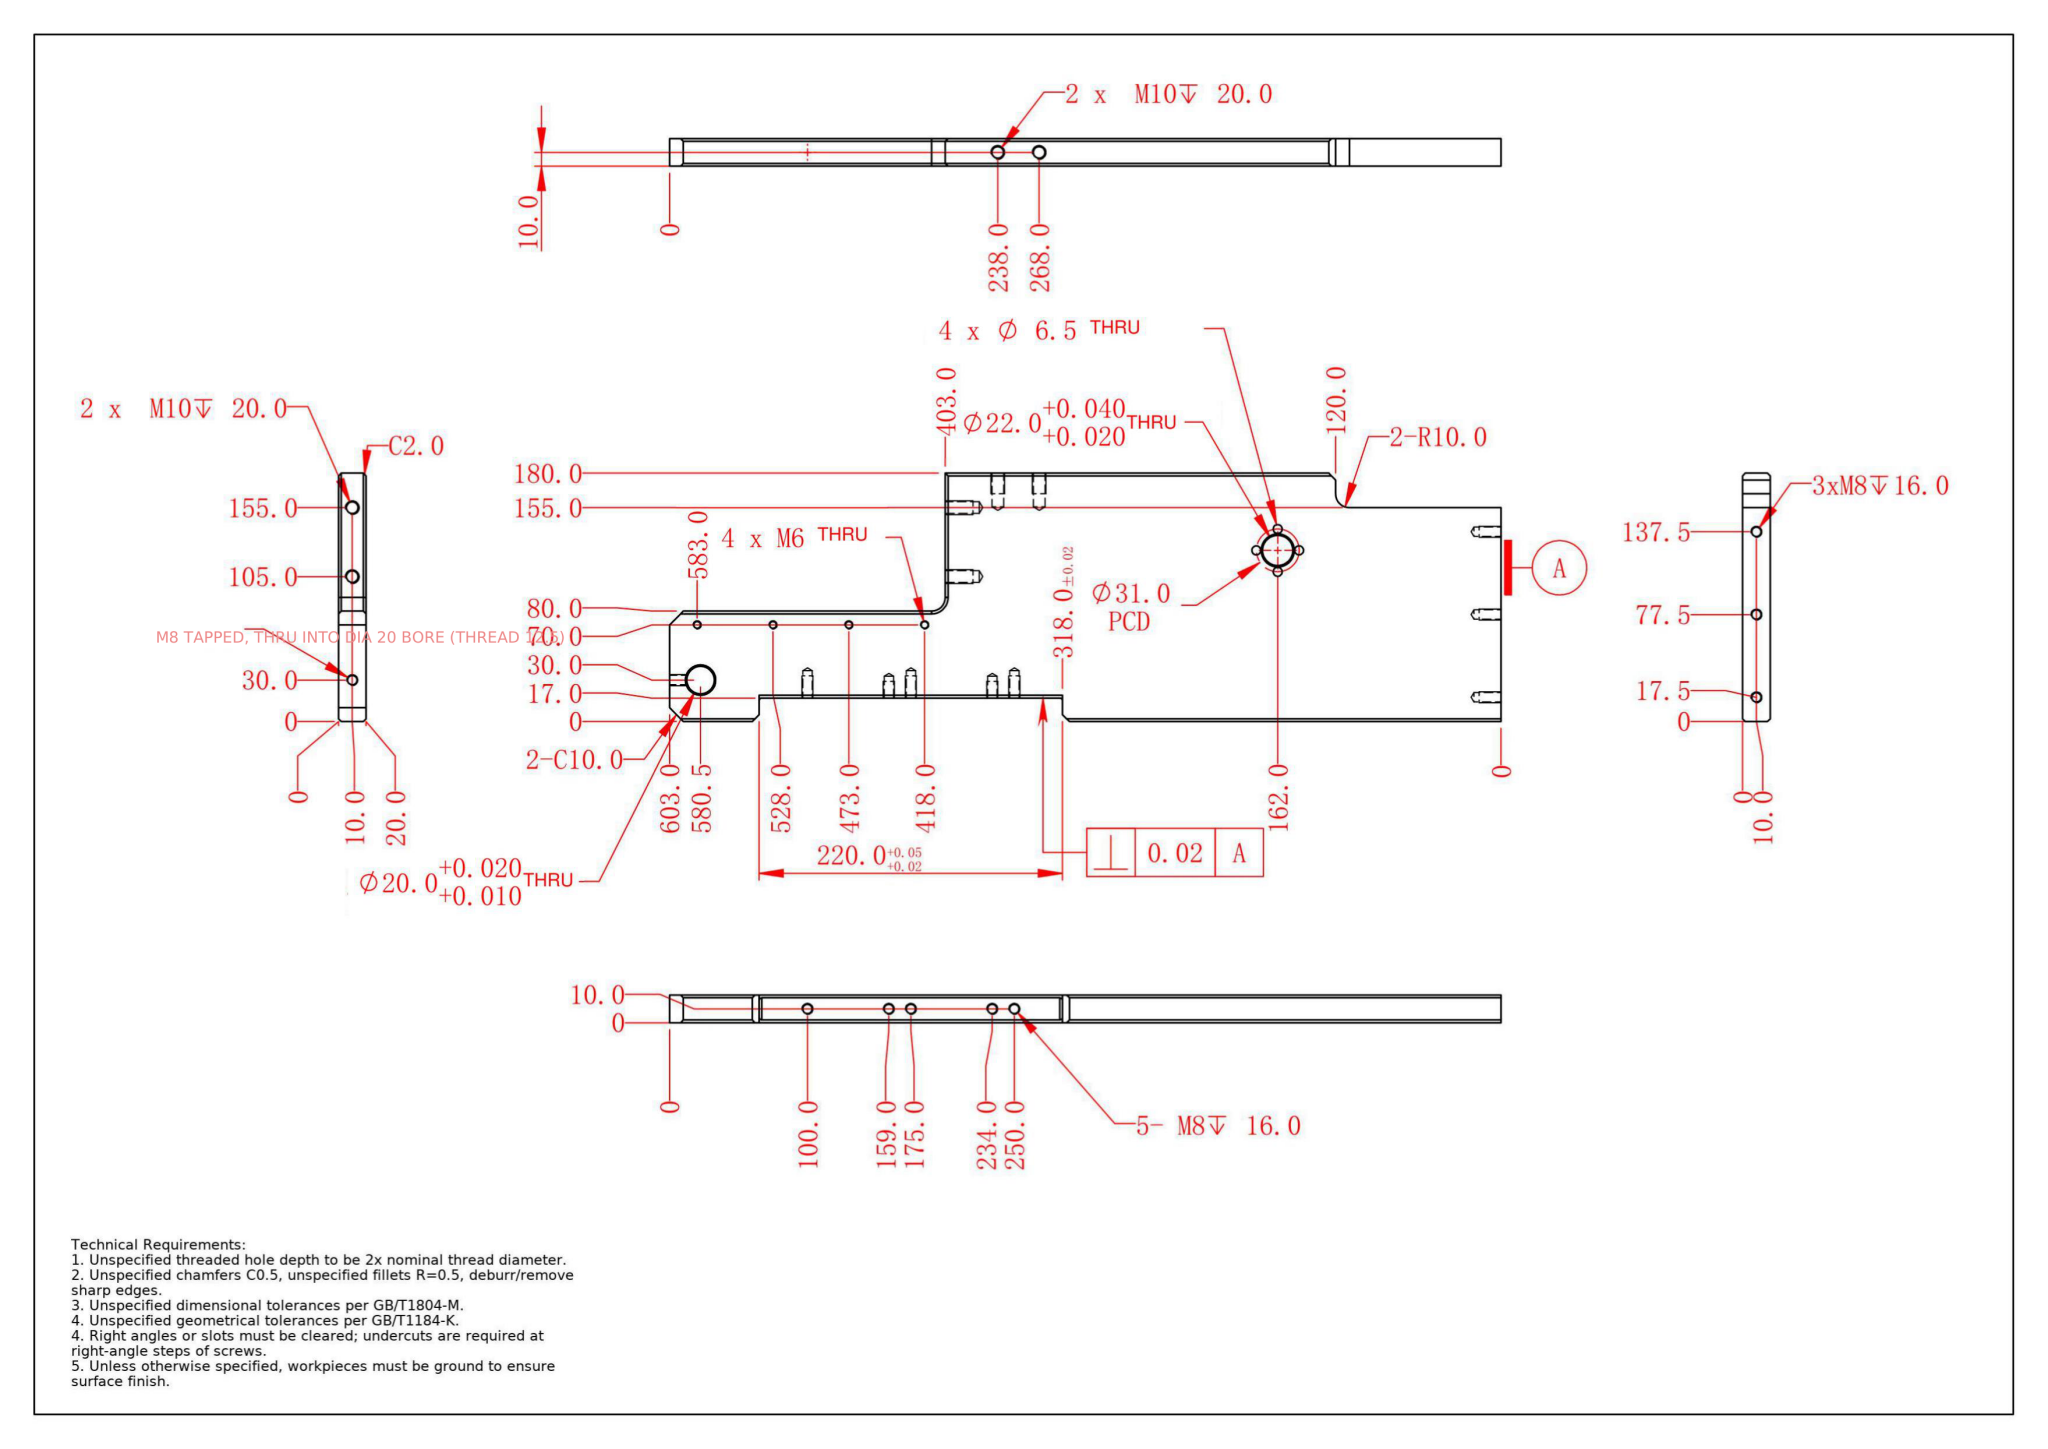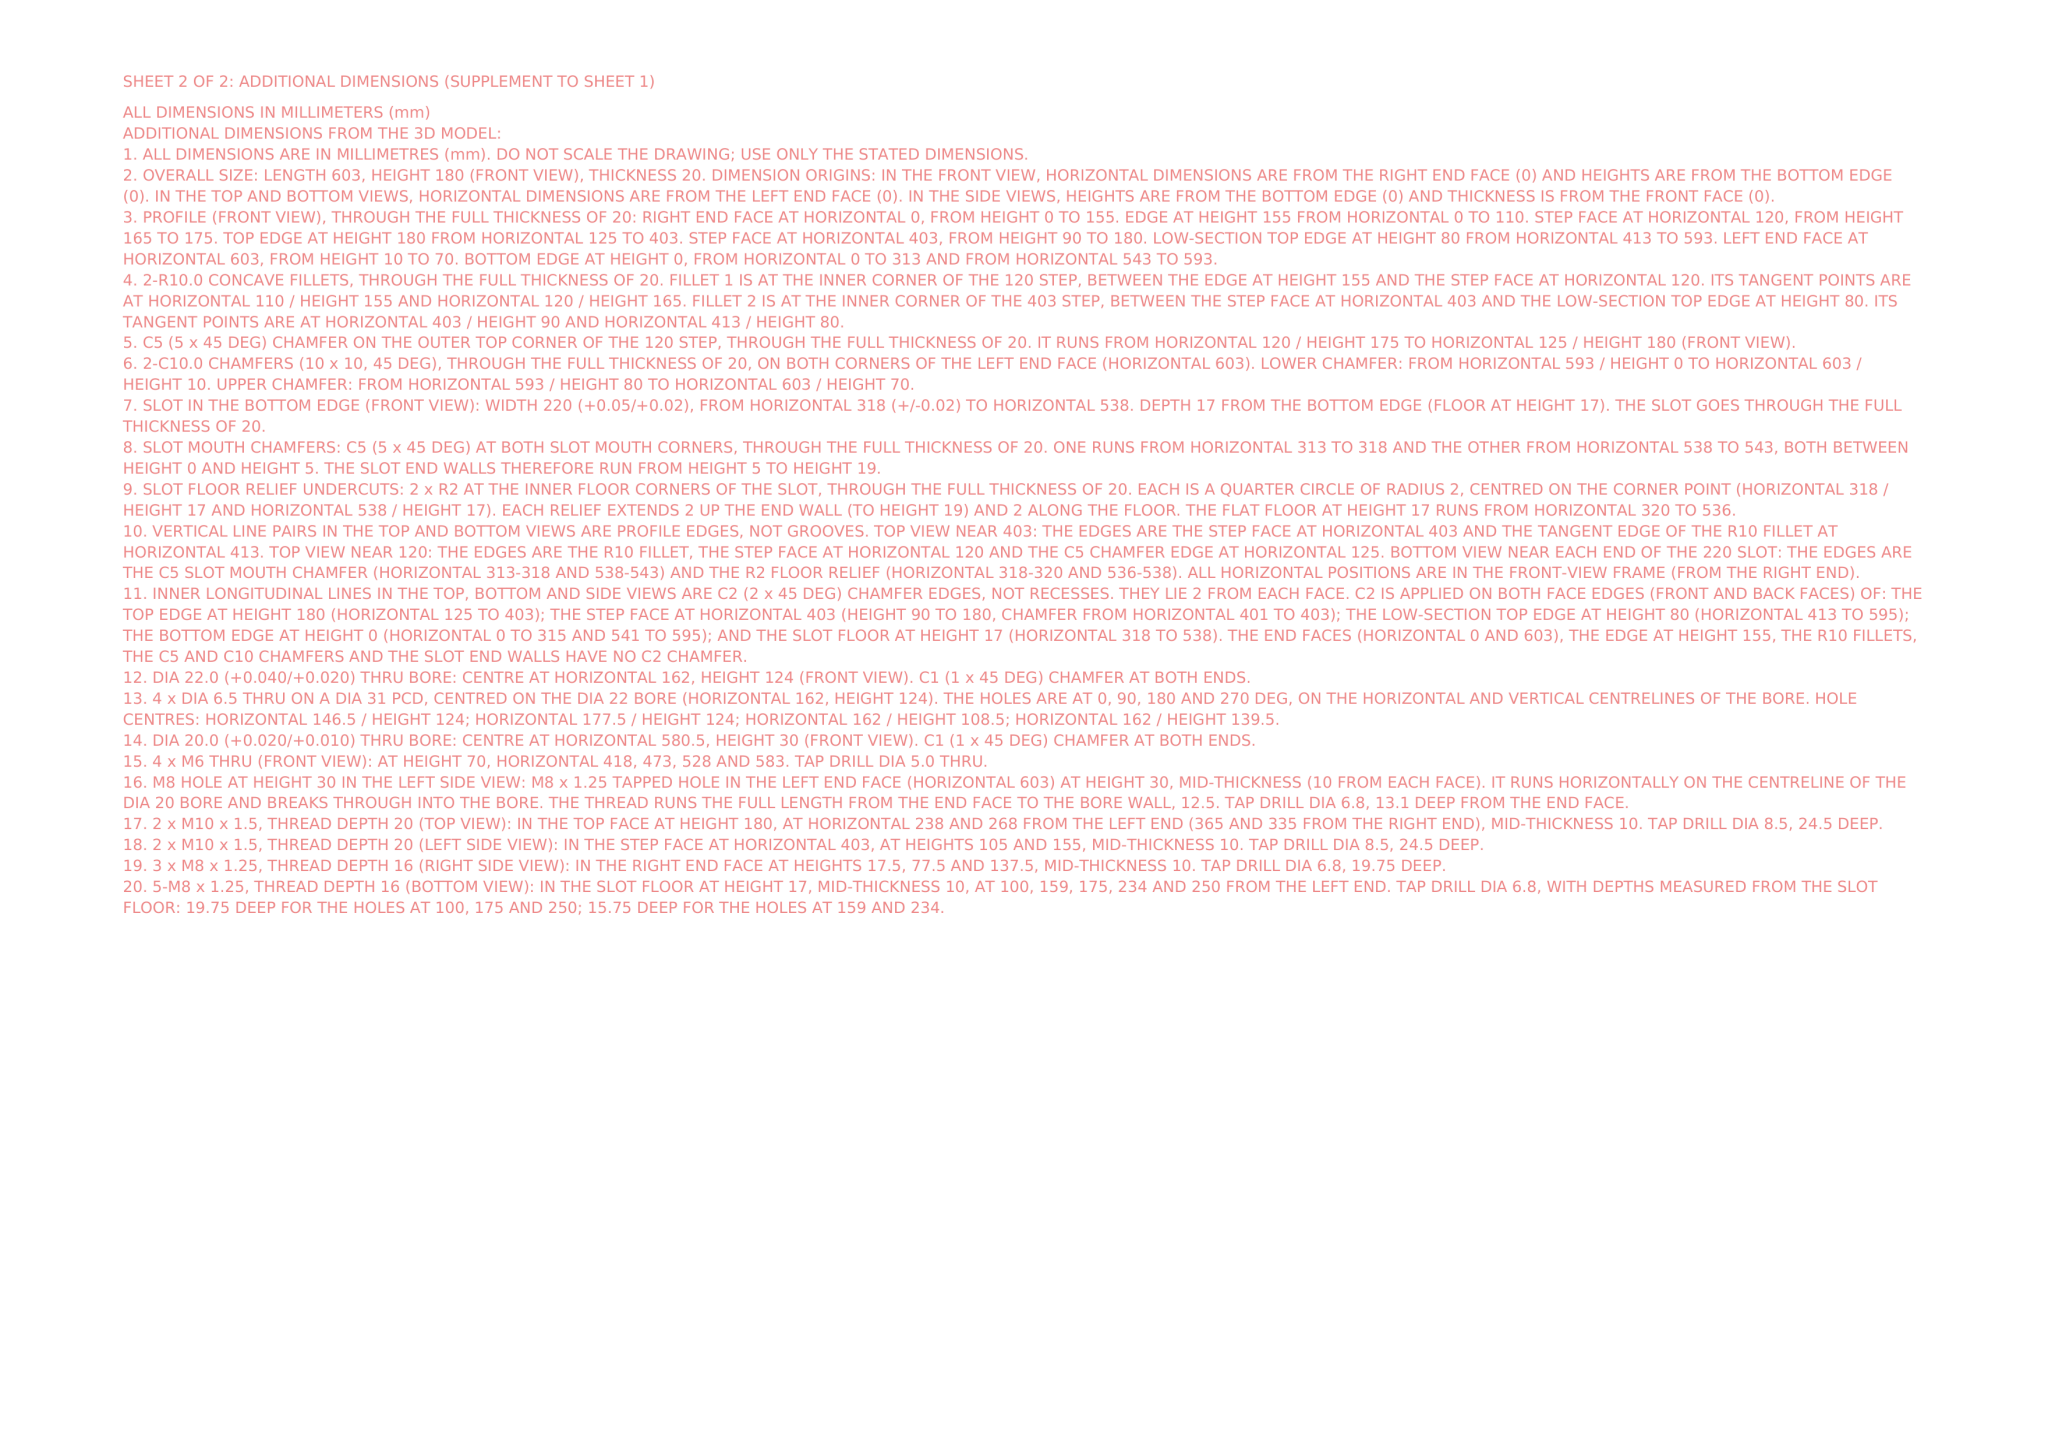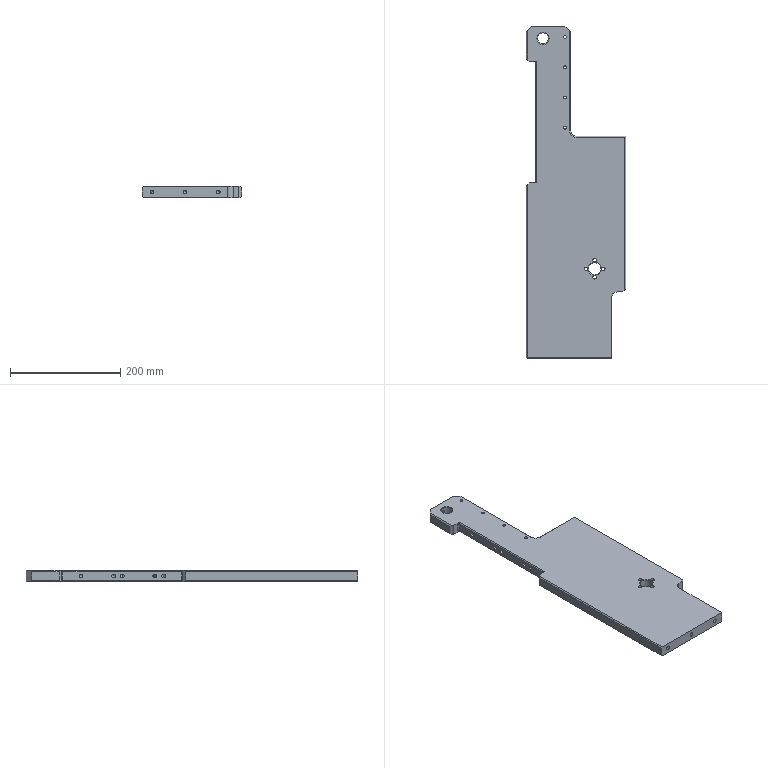Part | NX | mm | 1 solid | 115 faces | box 180 x 603 x 20 mm | volume 1599429 mm3 | cylinder 50 | cone 34 | plane 31 | commonest cylinder face diameters 6.8 x18 5 x8 8.5 x8 6.5 x8 20 x4 22 x2 4 x2